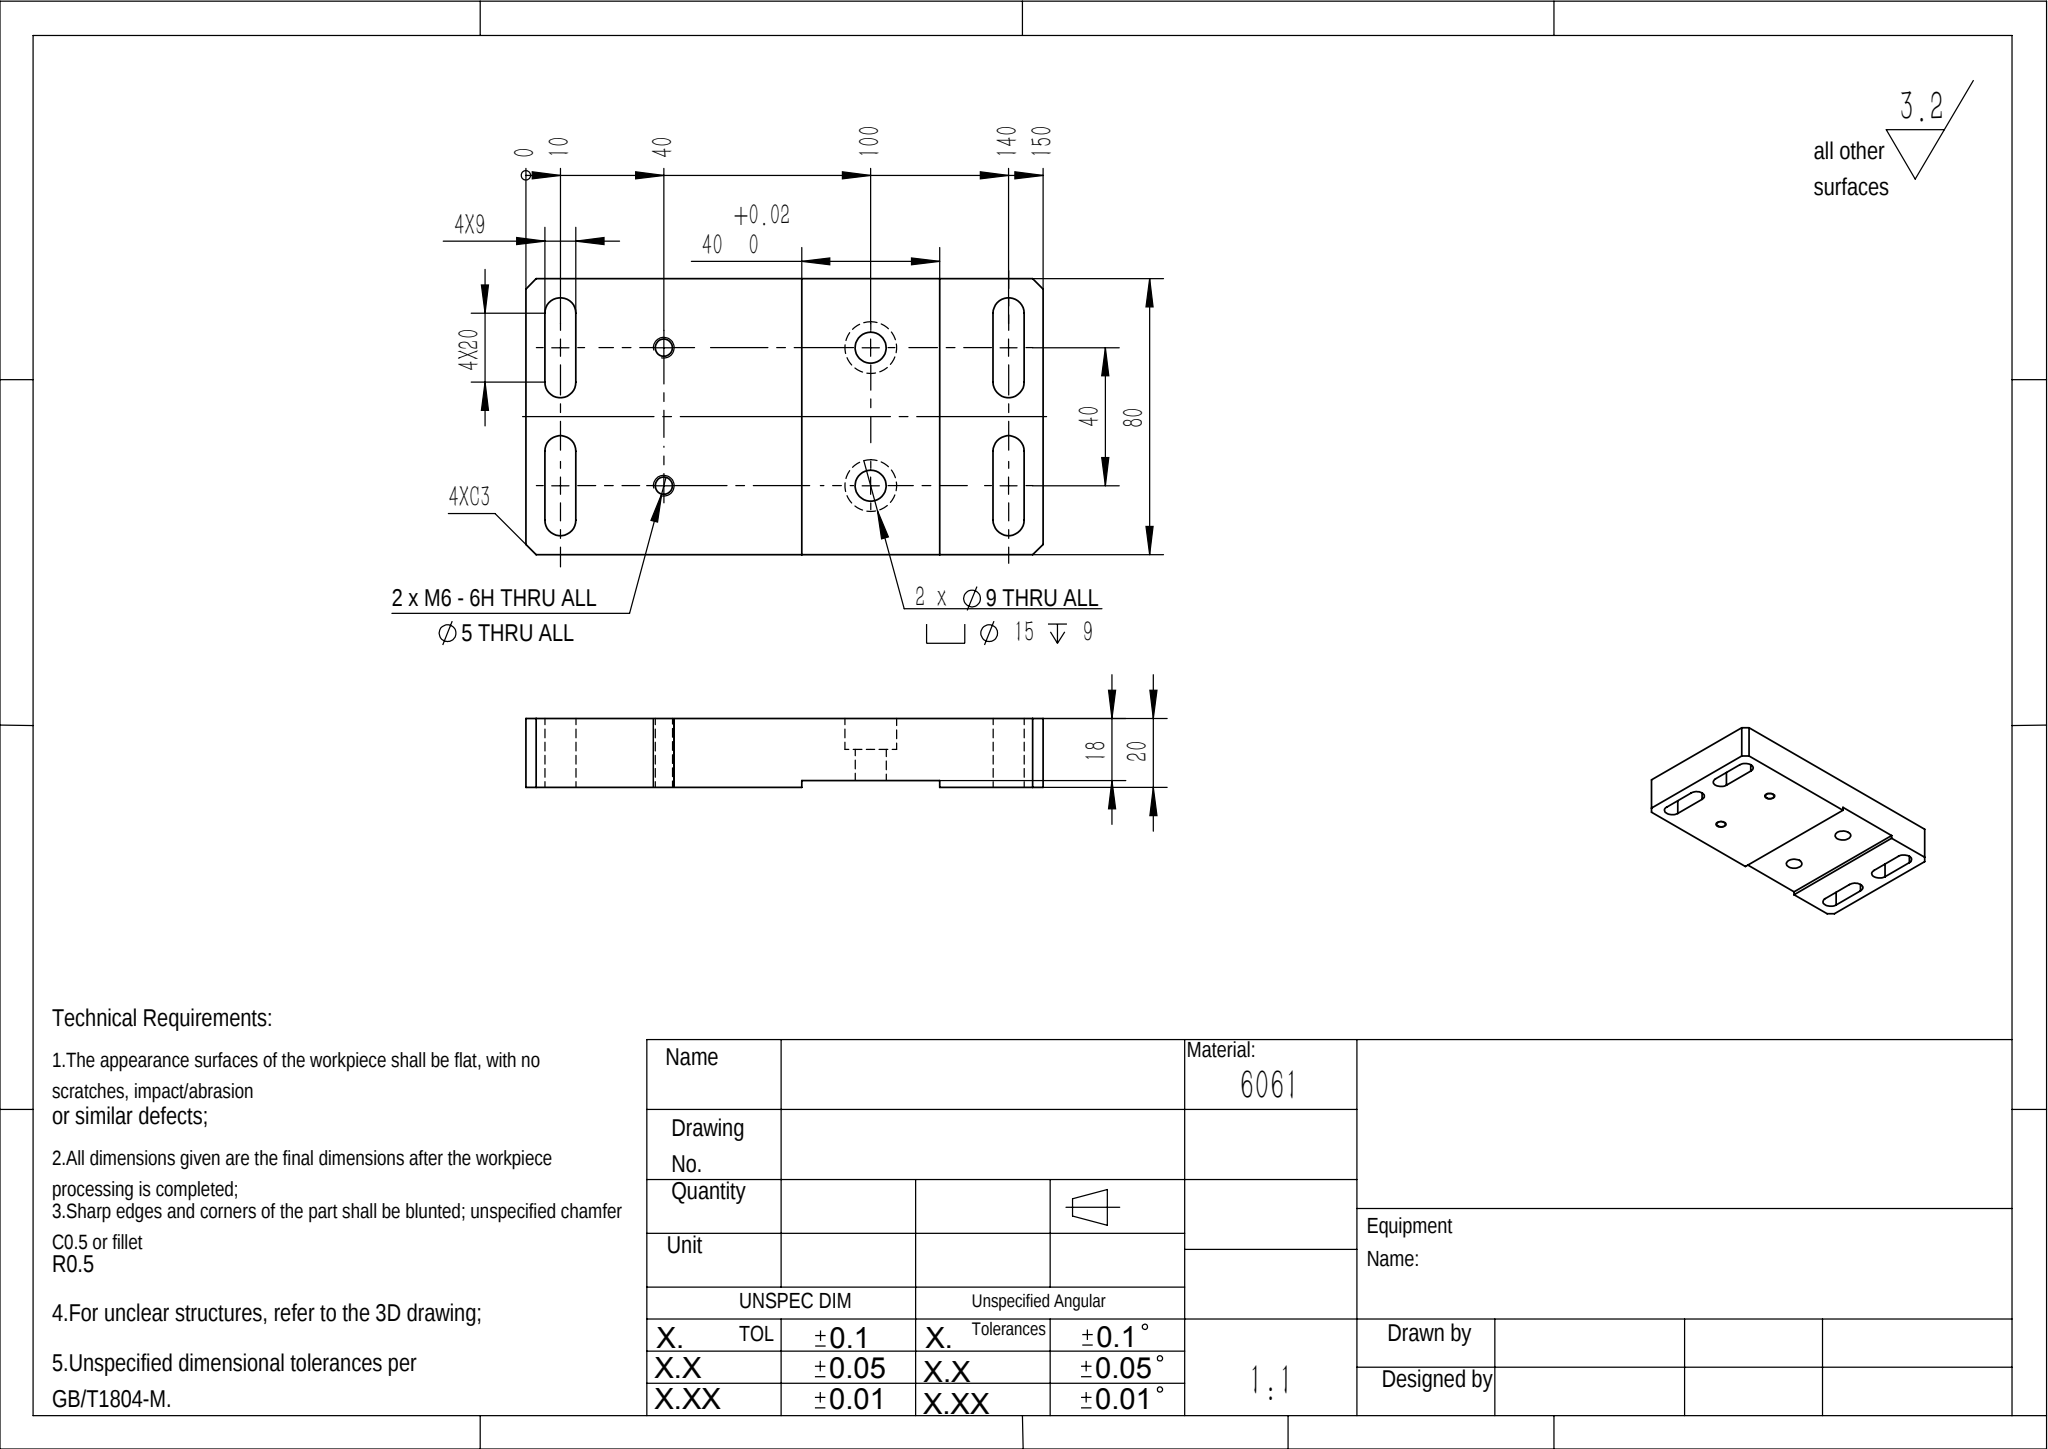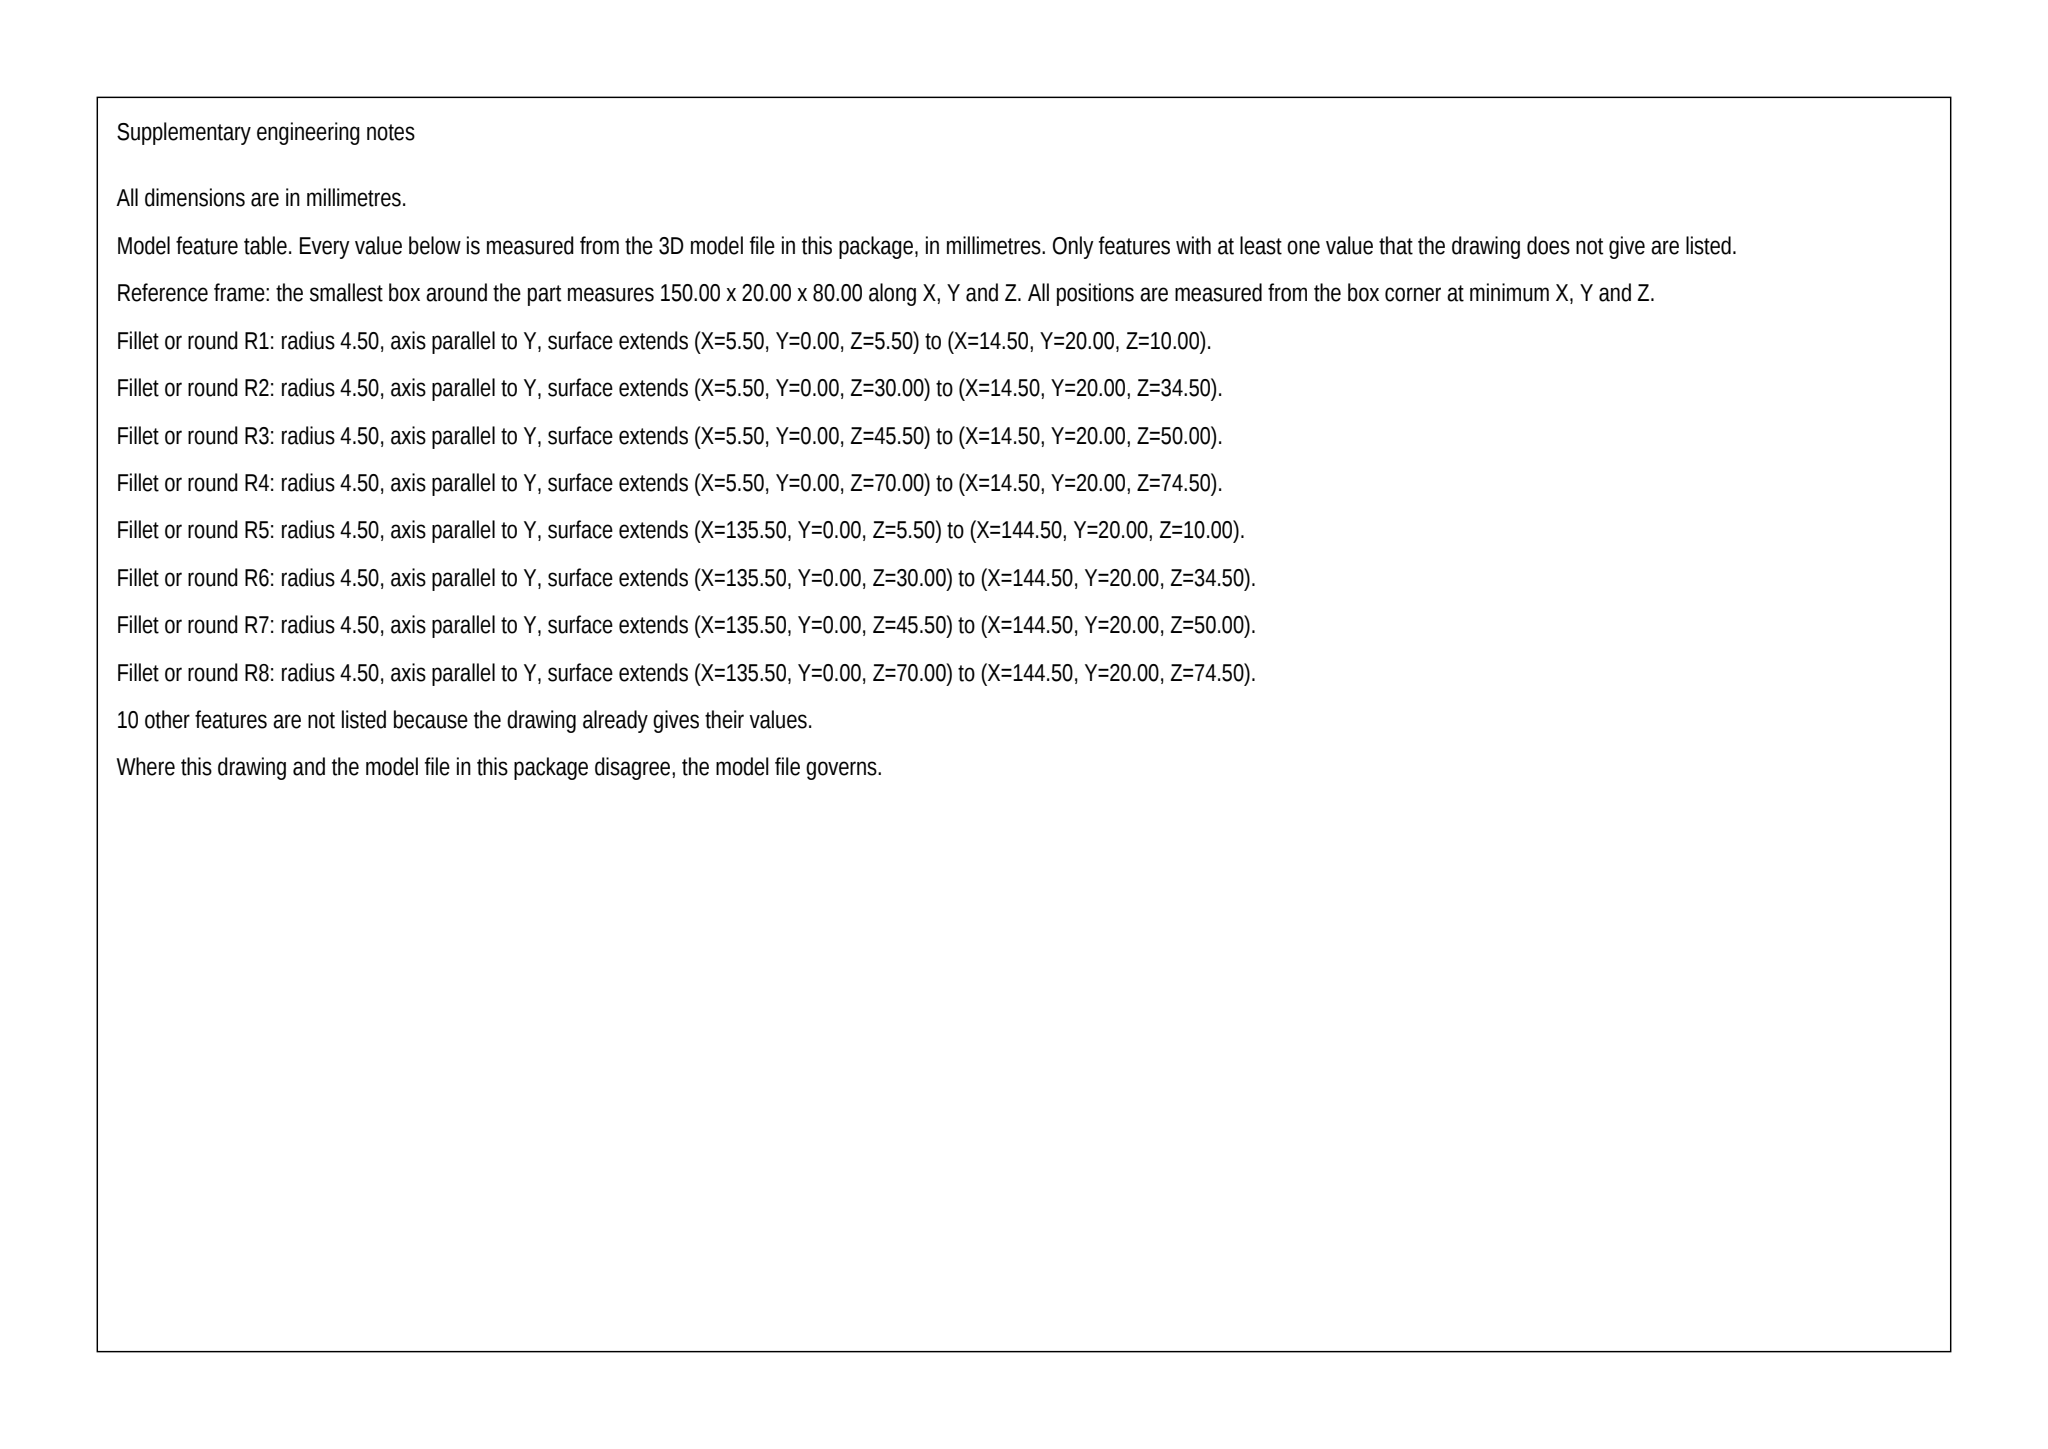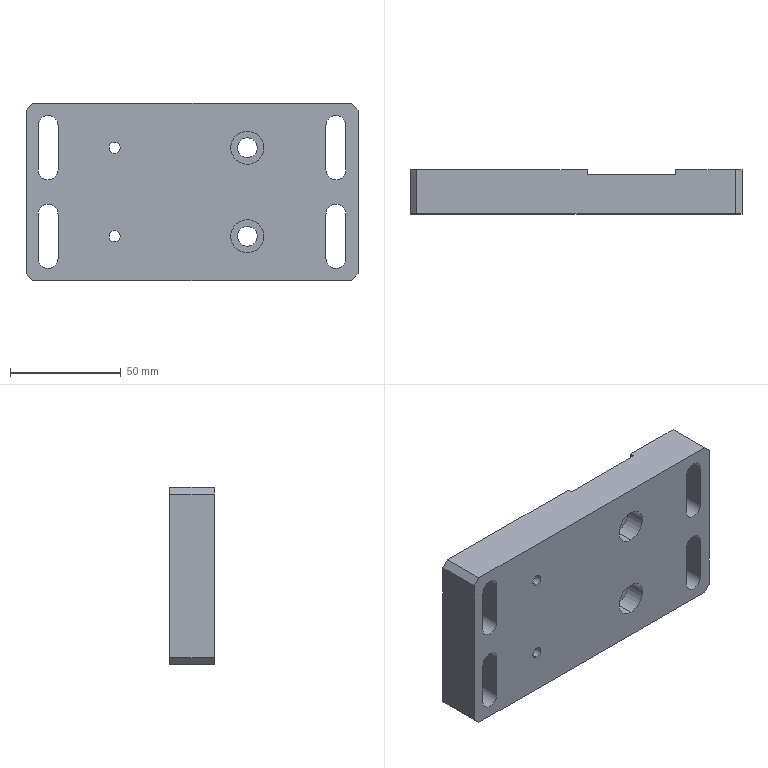Part | SolidWorks | mm | 1 solid | 48 faces | box 150 x 20 x 80 mm | volume 208639 mm3 | cylinder 24 | plane 24 | commonest cylinder face diameters 9 x16 5 x4 15 x4
Drawing notes:
SIDE VIEW: 2 DP STEP FROM X80 TO X120 OFF LH EDGE, FULL 80 WIDTH | from the solid: y-plane at 18.0 vs 20.0 top, bounded by x-planes 80.0 and 120.0; z extent 0-80
2 X M6-6H THRU AT 40 FROM LH EDGE; Ø5 IS TAP DRILL SIZE | from the solid: Ø5.0 cyls, axis y, length 20 (thru), at x=40, z=20 & z=60
2 X Ø9 THRU, CBORE Ø15 DP 9, AT 100 FROM LH EDGE | from the solid: Ø9 and Ø15 cyls at x=100, z=20 & z=60; bbox x=0..150, LH edge x=0
build123d program:
from build123d import *

# Parameters (mm, degrees)
SKETCH1_W                                         = 150
SKETCH1_H                                         = 80
BOSS_EXTRUDE1_DEPTH                               = 20
HOLE_SIZE_ACCORDING_TO_HEXAGON_SOCKET_D           = 9
HOLE_SIZE_ACCORDING_TO_HEXAGON_SOCKET_CBORE_D     = 15
HOLE_SIZE_ACCORDING_TO_HEXAGON_SOCKET_CBORE_DEPTH = 9
CUT_EXTRUDE2_DEPTH                                = 110.545
CHAMFER1_SIZE                                     = 3
SKETCH6_W                                         = 40
SKETCH6_H                                         = 80
CUT_EXTRUDE3_DEPTH                                = 2
M6_TAPPED_HOLE1_D                                 = 5


with BuildPart() as part:
    # Sketch1 → Boss-Extrude1 (new body)
    with BuildSketch(Plane(origin=(0, 0, 0), x_dir=(1, 0, 0), z_dir=(0, 1, 0))):
        with Locations((-25, 0)):
            Rectangle(SKETCH1_W, SKETCH1_H)
    extrude(amount=BOSS_EXTRUDE1_DEPTH)

    # Hole Size _ according to_ Hexagon Socket (through all)
    with Locations(Plane(origin=(0, 0, -20), x_dir=(0, 0, -1), z_dir=(0, -1, 0))):
        with Locations((0, 0), (-40, 0)):
            CounterBoreHole(HOLE_SIZE_ACCORDING_TO_HEXAGON_SOCKET_D / 2, HOLE_SIZE_ACCORDING_TO_HEXAGON_SOCKET_CBORE_D / 2, HOLE_SIZE_ACCORDING_TO_HEXAGON_SOCKET_CBORE_DEPTH)

    # Sketch5 → Cut-Extrude2 (cut, through all)
    with BuildSketch(Plane(origin=(0, 20, 0), x_dir=(1, 0, 0), z_dir=(0, 1, 0))):
        with BuildLine():
            Line((-94.5, 10), (-94.5, 30))
            ThreePointArc((-94.5, 30), (-90, 34.5), (-85.5, 30))
            Line((-85.5, 30), (-85.5, 10))
            ThreePointArc((-85.5, 10), (-90, 5.5), (-94.5, 10))
        make_face()
        with BuildLine():
            Line((-85.5, -10), (-85.5, -30))
            ThreePointArc((-85.5, -30), (-90, -34.5), (-94.5, -30))
            Line((-94.5, -30), (-94.5, -10))
            ThreePointArc((-94.5, -10), (-90, -5.5), (-85.5, -10))
        make_face()
        with BuildLine():
            Line((44.5, -10), (44.5, -30))
            ThreePointArc((44.5, -30), (40, -34.5), (35.5, -30))
            Line((35.5, -30), (35.5, -10))
            ThreePointArc((35.5, -10), (40, -5.5), (44.5, -10))
        make_face()
        with BuildLine():
            Line((35.5, 10), (35.5, 30))
            ThreePointArc((35.5, 30), (40, 34.5), (44.5, 30))
            Line((44.5, 30), (44.5, 10))
            ThreePointArc((44.5, 10), (40, 5.5), (35.5, 10))
        make_face()
    extrude(amount=-CUT_EXTRUDE2_DEPTH, mode=Mode.SUBTRACT)

    # Chamfer1
    chamfer1_edges = [part.edges().sort_by_distance(p)[0] for p in [
        (-100, 10, -40),
        (50, 10, -40),
        (50, 10, 40),
        (-100, 10, 40),
    ]]
    chamfer(chamfer1_edges, length=CHAMFER1_SIZE)

    # Sketch6 → Cut-Extrude3 (cut)
    with BuildSketch(Plane(origin=(0, 20, 0), x_dir=(1, 0, 0), z_dir=(0, 1, 0))):
        Rectangle(SKETCH6_W, SKETCH6_H)
    extrude(amount=-CUT_EXTRUDE3_DEPTH, mode=Mode.SUBTRACT)

    # M6 Tapped Hole1 (through all)
    with Locations(Plane(origin=(-60, 20, 20), x_dir=(0, 0, 1), z_dir=(0, 1, 0))):
        with Locations((0, 0), (-40, 0)):
            Hole(M6_TAPPED_HOLE1_D / 2)


solid = part.part